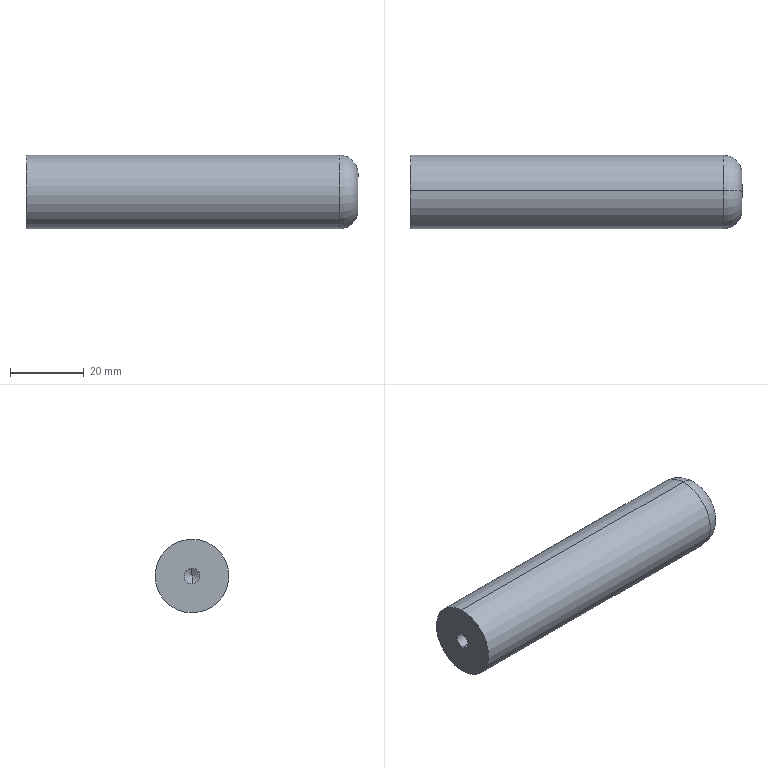Component | SolidWorks | AS-011-JG0104-1 | 1 solid | 10 faces | box 90 x 20 x 20 mm | volume 27775 mm3 | cylinder 4 | cone 2 | torus 2 | plane 2 | commonest cylinder face diameters 4.2 x2 20 x2
build123d program:
from build123d import *

# Parameters (mm, degrees)
SKETCH1_R             = 10
BOSS_EXTRUDE1_DEPTH   = 90
FILLET1_R             = 5
M5_TAPPED_HOLE1_D     = 4.2
M5_TAPPED_HOLE1_DEPTH = 14
M5_TAPPED_HOLE1_TIP   = 1.262


with BuildPart() as part:
    # Sketch1 → Boss-Extrude1 (new body)
    with BuildSketch(Plane.XY):
        with Locations(Location((0, 0, 0), (0, 0, 180))):
            Circle(SKETCH1_R)
    extrude(amount=BOSS_EXTRUDE1_DEPTH)

    # Fillet1
    fillet1_edges = [part.edges().sort_by_distance(p)[0] for p in [
        (10, 0, 90),
    ]]
    fillet(fillet1_edges, radius=FILLET1_R)

    # M5 Tapped Hole1
    with Locations(Plane(origin=(0, 0, 0), x_dir=(-1, 0, 0), z_dir=(0, 0, -1))):
        with Locations((0, 0)):
            Hole(M5_TAPPED_HOLE1_D / 2, depth=M5_TAPPED_HOLE1_DEPTH)
            with Locations((0, 0, -(M5_TAPPED_HOLE1_DEPTH + M5_TAPPED_HOLE1_TIP / 2))):  # 118° drill point
                Cone(0, M5_TAPPED_HOLE1_D / 2, M5_TAPPED_HOLE1_TIP, mode=Mode.SUBTRACT)


solid = part.part

# Placed as in the assembly
solid = solid.moved(Location((-51.5, -28, -112), (0, 90, 0)))
STEP:
#1=COLOUR_RGB('',0.7922,0.8196,0.9333);
#2=FILL_AREA_STYLE_COLOUR('',#1);
#3=FILL_AREA_STYLE('',(#2));
#4=SURFACE_STYLE_FILL_AREA(#3);
#5=SURFACE_SIDE_STYLE('',(#4));
#6=SURFACE_STYLE_USAGE(.BOTH.,#5);
#7=PRESENTATION_STYLE_ASSIGNMENT((#6));
#8=CARTESIAN_POINT('',(-1.476,-1.106,-4.492));
#9=VERTEX_POINT('',#8);
#10=CARTESIAN_POINT('',(-1.476,-1.099,-4.327));
#11=VERTEX_POINT('',#10);
#12=CARTESIAN_POINT('',(-1.476,-1.102,-4.409));
#13=DIRECTION('',(-1.,0.,0.));
#14=DIRECTION('',(0.,0.0408,0.9992));
#15=AXIS2_PLACEMENT_3D('',#12,#13,#14);
#16=CIRCLE('',#15,0.08268);
#17=EDGE_CURVE('',#9,#11,#16,.T.);
#18=ORIENTED_EDGE('',*,*,#17,.F.);
#19=CARTESIAN_POINT('',(-2.028,-1.106,-4.492));
#20=VERTEX_POINT('',#19);
#21=CARTESIAN_POINT('',(-2.028,-1.106,-4.492));
#22=DIRECTION('',(-1.,0.,0.));
#23=VECTOR('',#22,39.37);
#24=LINE('',#21,#23);
#25=EDGE_CURVE('',#9,#20,#24,.T.);
#26=ORIENTED_EDGE('',*,*,#25,.T.);
#27=CARTESIAN_POINT('',(-2.028,-1.099,-4.327));
#28=VERTEX_POINT('',#27);
#29=CARTESIAN_POINT('',(-2.028,-1.102,-4.409));
#30=DIRECTION('',(-1.,0.,0.));
#31=DIRECTION('',(0.,0.0408,0.9992));
#32=AXIS2_PLACEMENT_3D('',#29,#30,#31);
#33=CIRCLE('',#32,0.08268);
#34=EDGE_CURVE('',#20,#28,#33,.T.);
#35=ORIENTED_EDGE('',*,*,#34,.T.);
#36=CARTESIAN_POINT('',(-2.028,-1.099,-4.327));
#37=DIRECTION('',(-1.,0.,0.));
#38=VECTOR('',#37,39.37);
#39=LINE('',#36,#38);
#40=EDGE_CURVE('',#11,#28,#39,.T.);
#41=ORIENTED_EDGE('',*,*,#40,.F.);
#42=EDGE_LOOP('',(#18,#26,#35,#41));
#43=FACE_OUTER_BOUND('',#42,.T.);
#44=CARTESIAN_POINT('',(-2.028,-1.102,-4.409));
#45=DIRECTION('',(-1.,0.,0.));
#46=DIRECTION('',(0.,0.0408,0.9992));
#47=AXIS2_PLACEMENT_3D('',#44,#45,#46);
#48=CYLINDRICAL_SURFACE('',#47,0.08268);
#49=ADVANCED_FACE('',(#43),#48,.F.);
#50=CARTESIAN_POINT('',(-1.427,-1.102,-4.409));
#51=VERTEX_POINT('',#50);
#52=CARTESIAN_POINT('',(-1.476,-1.099,-4.327));
#53=DIRECTION('',(-0.515,0.03497,0.8565));
#54=VECTOR('',#53,39.37);
#55=LINE('',#52,#54);
#56=EDGE_CURVE('',#51,#11,#55,.T.);
#57=ORIENTED_EDGE('',*,*,#56,.F.);
#58=CARTESIAN_POINT('',(-1.476,-1.106,-4.492));
#59=DIRECTION('',(-0.515,-0.03497,-0.8565));
#60=VECTOR('',#59,39.37);
#61=LINE('',#58,#60);
#62=EDGE_CURVE('',#51,#9,#61,.T.);
#63=ORIENTED_EDGE('',*,*,#62,.T.);
#64=ORIENTED_EDGE('',*,*,#17,.T.);
#65=EDGE_LOOP('',(#57,#63,#64));
#66=FACE_OUTER_BOUND('',#65,.T.);
#67=CARTESIAN_POINT('',(-1.476,-1.102,-4.409));
#68=DIRECTION('',(-1.,0.,0.));
#69=DIRECTION('',(0.,0.0408,0.9992));
#70=AXIS2_PLACEMENT_3D('',#67,#68,#69);
#71=CONICAL_SURFACE('',#70,0.08268,1.03);
#72=ADVANCED_FACE('',(#66),#71,.F.);
#73=CARTESIAN_POINT('',(1.319,-1.086,-4.016));
#74=VERTEX_POINT('',#73);
#75=CARTESIAN_POINT('',(1.319,-1.118,-4.803));
#76=VERTEX_POINT('',#75);
#77=CARTESIAN_POINT('',(1.319,-1.102,-4.409));
#78=DIRECTION('',(-1.,0.,0.));
#79=DIRECTION('',(-0.,-0.0408,-0.9992));
#80=AXIS2_PLACEMENT_3D('',#77,#78,#79);
#81=CIRCLE('',#80,0.3937);
#82=EDGE_CURVE('',#74,#76,#81,.T.);
#83=ORIENTED_EDGE('',*,*,#82,.F.);
#84=CARTESIAN_POINT('',(1.516,-1.094,-4.213));
#85=VERTEX_POINT('',#84);
#86=CARTESIAN_POINT('',(1.319,-1.094,-4.213));
#87=DIRECTION('',(-0.,0.9992,-0.0408));
#88=DIRECTION('',(0.,0.0408,0.9992));
#89=AXIS2_PLACEMENT_3D('',#86,#87,#88);
#90=CIRCLE('',#89,0.1969);
#91=EDGE_CURVE('',#74,#85,#90,.T.);
#92=ORIENTED_EDGE('',*,*,#91,.T.);
#93=CARTESIAN_POINT('',(1.516,-1.11,-4.606));
#94=VERTEX_POINT('',#93);
#95=CARTESIAN_POINT('',(1.516,-1.102,-4.409));
#96=DIRECTION('',(1.,-0.,-0.));
#97=DIRECTION('',(-0.,-0.0408,-0.9992));
#98=AXIS2_PLACEMENT_3D('',#95,#96,#97);
#99=CIRCLE('',#98,0.1969);
#100=EDGE_CURVE('',#94,#85,#99,.T.);
#101=ORIENTED_EDGE('',*,*,#100,.F.);
#102=CARTESIAN_POINT('',(1.319,-1.11,-4.606));
#103=DIRECTION('',(0.,-0.9992,0.0408));
#104=DIRECTION('',(0.,-0.0408,-0.9992));
#105=AXIS2_PLACEMENT_3D('',#102,#103,#104);
#106=CIRCLE('',#105,0.1969);
#107=EDGE_CURVE('',#76,#94,#106,.T.);
#108=ORIENTED_EDGE('',*,*,#107,.F.);
#109=EDGE_LOOP('',(#83,#92,#101,#108));
#110=FACE_OUTER_BOUND('',#109,.T.);
#111=CARTESIAN_POINT('',(1.319,-1.102,-4.409));
#112=DIRECTION('',(1.,-0.,-0.));
#113=DIRECTION('',(-0.,-0.0408,-0.9992));
#114=AXIS2_PLACEMENT_3D('',#111,#112,#113);
#115=TOROIDAL_SURFACE('',#114,0.1969,0.1969);
#116=ADVANCED_FACE('',(#110),#115,.T.);
#117=ORIENTED_EDGE('',*,*,#82,.T.);
#118=CARTESIAN_POINT('',(-2.028,-1.118,-4.803));
#119=VERTEX_POINT('',#118);
#120=CARTESIAN_POINT('',(1.516,-1.118,-4.803));
#121=DIRECTION('',(-1.,0.,0.));
#122=VECTOR('',#121,39.37);
#123=LINE('',#120,#122);
#124=EDGE_CURVE('',#76,#119,#123,.T.);
#125=ORIENTED_EDGE('',*,*,#124,.T.);
#126=CARTESIAN_POINT('',(-2.028,-1.086,-4.016));
#127=VERTEX_POINT('',#126);
#128=CARTESIAN_POINT('',(-2.028,-1.102,-4.409));
#129=DIRECTION('',(1.,-0.,-0.));
#130=DIRECTION('',(-0.,-0.0408,-0.9992));
#131=AXIS2_PLACEMENT_3D('',#128,#129,#130);
#132=CIRCLE('',#131,0.3937);
#133=EDGE_CURVE('',#119,#127,#132,.T.);
#134=ORIENTED_EDGE('',*,*,#133,.T.);
#135=CARTESIAN_POINT('',(1.516,-1.086,-4.016));
#136=DIRECTION('',(-1.,0.,0.));
#137=VECTOR('',#136,39.37);
#138=LINE('',#135,#137);
#139=EDGE_CURVE('',#74,#127,#138,.T.);
#140=ORIENTED_EDGE('',*,*,#139,.F.);
#141=EDGE_LOOP('',(#117,#125,#134,#140));
#142=FACE_OUTER_BOUND('',#141,.T.);
#143=CARTESIAN_POINT('',(1.516,-1.102,-4.409));
#144=DIRECTION('',(-1.,0.,0.));
#145=DIRECTION('',(0.,0.0408,0.9992));
#146=AXIS2_PLACEMENT_3D('',#143,#144,#145);
#147=CYLINDRICAL_SURFACE('',#146,0.3937);
#148=ADVANCED_FACE('',(#142),#147,.T.);
#149=ORIENTED_EDGE('',*,*,#124,.F.);
#150=CARTESIAN_POINT('',(1.319,-1.102,-4.409));
#151=DIRECTION('',(-1.,0.,0.));
#152=DIRECTION('',(-0.,-0.0408,-0.9992));
#153=AXIS2_PLACEMENT_3D('',#150,#151,#152);
#154=CIRCLE('',#153,0.3937);
#155=EDGE_CURVE('',#76,#74,#154,.T.);
#156=ORIENTED_EDGE('',*,*,#155,.T.);
#157=ORIENTED_EDGE('',*,*,#139,.T.);
#158=CARTESIAN_POINT('',(-2.028,-1.102,-4.409));
#159=DIRECTION('',(1.,-0.,-0.));
#160=DIRECTION('',(-0.,-0.0408,-0.9992));
#161=AXIS2_PLACEMENT_3D('',#158,#159,#160);
#162=CIRCLE('',#161,0.3937);
#163=EDGE_CURVE('',#127,#119,#162,.T.);
#164=ORIENTED_EDGE('',*,*,#163,.T.);
#165=EDGE_LOOP('',(#149,#156,#157,#164));
#166=FACE_OUTER_BOUND('',#165,.T.);
#167=CARTESIAN_POINT('',(1.516,-1.102,-4.409));
#168=DIRECTION('',(-1.,0.,0.));
#169=DIRECTION('',(0.,0.0408,0.9992));
#170=AXIS2_PLACEMENT_3D('',#167,#168,#169);
#171=CYLINDRICAL_SURFACE('',#170,0.3937);
#172=ADVANCED_FACE('',(#166),#171,.T.);
#173=ORIENTED_EDGE('',*,*,#100,.T.);
#174=CARTESIAN_POINT('',(1.516,-1.102,-4.409));
#175=DIRECTION('',(1.,-0.,-0.));
#176=DIRECTION('',(-0.,-0.0408,-0.9992));
#177=AXIS2_PLACEMENT_3D('',#174,#175,#176);
#178=CIRCLE('',#177,0.1969);
#179=EDGE_CURVE('',#85,#94,#178,.T.);
#180=ORIENTED_EDGE('',*,*,#179,.T.);
#181=EDGE_LOOP('',(#173,#180));
#182=FACE_OUTER_BOUND('',#181,.T.);
#183=CARTESIAN_POINT('',(1.516,-1.102,-4.409));
#184=DIRECTION('',(1.,-0.,-0.));
#185=DIRECTION('',(-0.,-0.0408,-0.9992));
#186=AXIS2_PLACEMENT_3D('',#183,#184,#185);
#187=PLANE('',#186);
#188=ADVANCED_FACE('',(#182),#187,.T.);
#189=CARTESIAN_POINT('',(-2.028,-1.102,-4.409));
#190=DIRECTION('',(-1.,0.,0.));
#191=DIRECTION('',(0.,0.0408,0.9992));
#192=AXIS2_PLACEMENT_3D('',#189,#190,#191);
#193=CIRCLE('',#192,0.08268);
#194=EDGE_CURVE('',#28,#20,#193,.T.);
#195=ORIENTED_EDGE('',*,*,#194,.F.);
#196=ORIENTED_EDGE('',*,*,#34,.F.);
#197=EDGE_LOOP('',(#195,#196));
#198=FACE_BOUND('',#197,.T.);
#199=ORIENTED_EDGE('',*,*,#163,.F.);
#200=ORIENTED_EDGE('',*,*,#133,.F.);
#201=EDGE_LOOP('',(#199,#200));
#202=FACE_OUTER_BOUND('',#201,.T.);
#203=CARTESIAN_POINT('',(-2.028,-1.102,-4.409));
#204=DIRECTION('',(1.,-0.,-0.));
#205=DIRECTION('',(-0.,-0.0408,-0.9992));
#206=AXIS2_PLACEMENT_3D('',#203,#204,#205);
#207=PLANE('',#206);
#208=ADVANCED_FACE('',(#198,#202),#207,.F.);
#209=ORIENTED_EDGE('',*,*,#91,.F.);
#210=ORIENTED_EDGE('',*,*,#155,.F.);
#211=ORIENTED_EDGE('',*,*,#107,.T.);
#212=ORIENTED_EDGE('',*,*,#179,.F.);
#213=EDGE_LOOP('',(#209,#210,#211,#212));
#214=FACE_OUTER_BOUND('',#213,.T.);
#215=CARTESIAN_POINT('',(1.319,-1.102,-4.409));
#216=DIRECTION('',(1.,-0.,-0.));
#217=DIRECTION('',(-0.,-0.0408,-0.9992));
#218=AXIS2_PLACEMENT_3D('',#215,#216,#217);
#219=TOROIDAL_SURFACE('',#218,0.1969,0.1969);
#220=ADVANCED_FACE('',(#214),#219,.T.);
#221=ORIENTED_EDGE('',*,*,#62,.F.);
#222=ORIENTED_EDGE('',*,*,#56,.T.);
#223=CARTESIAN_POINT('',(-1.476,-1.102,-4.409));
#224=DIRECTION('',(-1.,0.,0.));
#225=DIRECTION('',(0.,0.0408,0.9992));
#226=AXIS2_PLACEMENT_3D('',#223,#224,#225);
#227=CIRCLE('',#226,0.08268);
#228=EDGE_CURVE('',#11,#9,#227,.T.);
#229=ORIENTED_EDGE('',*,*,#228,.T.);
#230=EDGE_LOOP('',(#221,#222,#229));
#231=FACE_OUTER_BOUND('',#230,.T.);
#232=CARTESIAN_POINT('',(-1.476,-1.102,-4.409));
#233=DIRECTION('',(-1.,0.,0.));
#234=DIRECTION('',(0.,0.0408,0.9992));
#235=AXIS2_PLACEMENT_3D('',#232,#233,#234);
#236=CONICAL_SURFACE('',#235,0.08268,1.03);
#237=ADVANCED_FACE('',(#231),#236,.F.);
#238=ORIENTED_EDGE('',*,*,#25,.F.);
#239=ORIENTED_EDGE('',*,*,#228,.F.);
#240=ORIENTED_EDGE('',*,*,#40,.T.);
#241=ORIENTED_EDGE('',*,*,#194,.T.);
#242=EDGE_LOOP('',(#238,#239,#240,#241));
#243=FACE_OUTER_BOUND('',#242,.T.);
#244=CARTESIAN_POINT('',(-2.028,-1.102,-4.409));
#245=DIRECTION('',(-1.,0.,0.));
#246=DIRECTION('',(0.,0.0408,0.9992));
#247=AXIS2_PLACEMENT_3D('',#244,#245,#246);
#248=CYLINDRICAL_SURFACE('',#247,0.08268);
#249=ADVANCED_FACE('',(#243),#248,.F.);
#250=CLOSED_SHELL('',(#49,#72,#116,#148,#172,#188,#208,#220,#237,#249));
#251=MANIFOLD_SOLID_BREP('',#250);
#252=STYLED_ITEM('',(#7),#251);
#253=(LENGTH_UNIT()NAMED_UNIT(*)SI_UNIT($,.METRE.));
#254=LENGTH_MEASURE_WITH_UNIT(LENGTH_MEASURE(0.0254),#253);
#255=DIMENSIONAL_EXPONENTS(1.,0.,0.,0.,0.,0.,0.);
#256=(CONVERSION_BASED_UNIT('',#254)LENGTH_UNIT()NAMED_UNIT(#255));
#257=UNCERTAINTY_MEASURE_WITH_UNIT(LENGTH_MEASURE(0.00001),#256,'','');
#258=(NAMED_UNIT(*)PLANE_ANGLE_UNIT()SI_UNIT($,.RADIAN.));
#259=(NAMED_UNIT(*)SI_UNIT($,.STERADIAN.)SOLID_ANGLE_UNIT());
#260=(GEOMETRIC_REPRESENTATION_CONTEXT(3)GLOBAL_UNCERTAINTY_ASSIGNED_CONTEXT((#257))GLOBAL_UNIT_ASSIGNED_CONTEXT((#256,#258,#259))REPRESENTATION_CONTEXT('',''));
#261=MECHANICAL_DESIGN_GEOMETRIC_PRESENTATION_REPRESENTATION('',(#252),#260);
#262=PRESENTATION_LAYER_ASSIGNMENT('','',(#252));
#263=CARTESIAN_POINT('',(0.,0.,0.));
#264=DIRECTION('',(0.,0.,1.));
#265=DIRECTION('',(1.,0.,0.));
#266=AXIS2_PLACEMENT_3D('',#263,#264,#265);
#267=(LENGTH_UNIT()NAMED_UNIT(*)SI_UNIT($,.METRE.));
#268=LENGTH_MEASURE_WITH_UNIT(LENGTH_MEASURE(0.0254),#267);
#269=DIMENSIONAL_EXPONENTS(1.,0.,0.,0.,0.,0.,0.);
#270=(CONVERSION_BASED_UNIT('',#268)LENGTH_UNIT()NAMED_UNIT(#269));
#271=UNCERTAINTY_MEASURE_WITH_UNIT(LENGTH_MEASURE(0.00001),#270,'','');
#272=(NAMED_UNIT(*)PLANE_ANGLE_UNIT()SI_UNIT($,.RADIAN.));
#273=(NAMED_UNIT(*)SI_UNIT($,.STERADIAN.)SOLID_ANGLE_UNIT());
#274=(GEOMETRIC_REPRESENTATION_CONTEXT(3)GLOBAL_UNCERTAINTY_ASSIGNED_CONTEXT((#271))GLOBAL_UNIT_ASSIGNED_CONTEXT((#270,#272,#273))REPRESENTATION_CONTEXT('',''));
#275=ADVANCED_BREP_SHAPE_REPRESENTATION('',(#251,#266),#274);